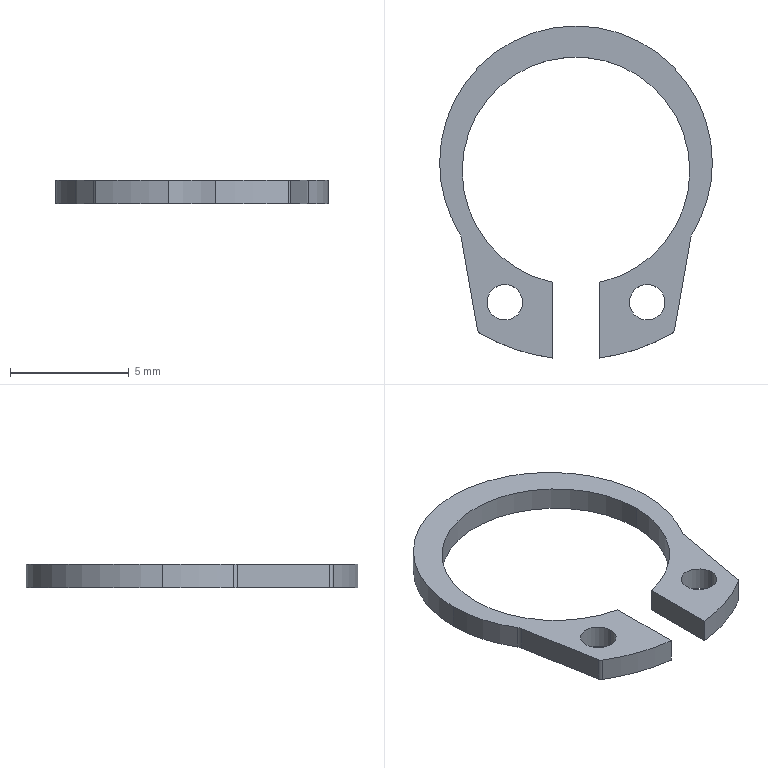Component | SolidWorks | ShaftRetainingRing_10-1 | 1 solid | 22 faces | box 11.5 x 14 x 1 mm | volume 46 mm3 | cylinder 16 | plane 6 | commonest cylinder face diameters 1.5 x4 9.6 x3 11.5 x3 15.9 x2 0.4 x2 1 x2 | material Purchased Part
STEP:
#1=COLOUR_RGB('',0.7922,0.8196,0.9333);
#2=FILL_AREA_STYLE_COLOUR('',#1);
#3=FILL_AREA_STYLE('',(#2));
#4=SURFACE_STYLE_FILL_AREA(#3);
#5=SURFACE_SIDE_STYLE('',(#4));
#6=SURFACE_STYLE_USAGE(.BOTH.,#5);
#7=PRESENTATION_STYLE_ASSIGNMENT((#6));
#8=CARTESIAN_POINT('',(-0.07087,-0.9843,0.9055));
#9=VERTEX_POINT('',#8);
#10=CARTESIAN_POINT('',(0.07874,-1.169,0.9055));
#11=VERTEX_POINT('',#10);
#12=CARTESIAN_POINT('',(0.1181,-0.9843,0.9055));
#13=DIRECTION('',(0.,0.,1.));
#14=DIRECTION('',(-1.,0.,0.));
#15=AXIS2_PLACEMENT_3D('',#12,#13,#14);
#16=CIRCLE('',#15,0.189);
#17=EDGE_CURVE('',#9,#11,#16,.T.);
#18=ORIENTED_EDGE('',*,*,#17,.F.);
#19=CARTESIAN_POINT('',(-0.07087,-0.9843,0.9449));
#20=VERTEX_POINT('',#19);
#21=CARTESIAN_POINT('',(-0.07087,-0.9843,0.9055));
#22=DIRECTION('',(0.,0.,1.));
#23=VECTOR('',#22,39.37);
#24=LINE('',#21,#23);
#25=EDGE_CURVE('',#9,#20,#24,.T.);
#26=ORIENTED_EDGE('',*,*,#25,.T.);
#27=CARTESIAN_POINT('',(0.07874,-1.169,0.9449));
#28=VERTEX_POINT('',#27);
#29=CARTESIAN_POINT('',(0.1181,-0.9843,0.9449));
#30=DIRECTION('',(0.,0.,-1.));
#31=DIRECTION('',(-1.,0.,0.));
#32=AXIS2_PLACEMENT_3D('',#29,#30,#31);
#33=CIRCLE('',#32,0.189);
#34=EDGE_CURVE('',#28,#20,#33,.T.);
#35=ORIENTED_EDGE('',*,*,#34,.F.);
#36=CARTESIAN_POINT('',(0.07874,-1.169,0.9055));
#37=DIRECTION('',(0.,0.,1.));
#38=VECTOR('',#37,39.37);
#39=LINE('',#36,#38);
#40=EDGE_CURVE('',#11,#28,#39,.T.);
#41=ORIENTED_EDGE('',*,*,#40,.F.);
#42=EDGE_LOOP('',(#18,#26,#35,#41));
#43=FACE_OUTER_BOUND('',#42,.T.);
#44=CARTESIAN_POINT('',(0.1181,-0.9843,0.9055));
#45=DIRECTION('',(0.,0.,1.));
#46=DIRECTION('',(1.,0.,0.));
#47=AXIS2_PLACEMENT_3D('',#44,#45,#46);
#48=CYLINDRICAL_SURFACE('',#47,0.189);
#49=ADVANCED_FACE('',(#43),#48,.F.);
#50=ORIENTED_EDGE('',*,*,#25,.F.);
#51=CARTESIAN_POINT('',(0.3071,-0.9843,0.9055));
#52=VERTEX_POINT('',#51);
#53=CARTESIAN_POINT('',(0.1181,-0.9843,0.9055));
#54=DIRECTION('',(0.,0.,1.));
#55=DIRECTION('',(-1.,0.,0.));
#56=AXIS2_PLACEMENT_3D('',#53,#54,#55);
#57=CIRCLE('',#56,0.189);
#58=EDGE_CURVE('',#52,#9,#57,.T.);
#59=ORIENTED_EDGE('',*,*,#58,.F.);
#60=CARTESIAN_POINT('',(0.3071,-0.9843,0.9449));
#61=VERTEX_POINT('',#60);
#62=CARTESIAN_POINT('',(0.3071,-0.9843,0.9055));
#63=DIRECTION('',(0.,0.,1.));
#64=VECTOR('',#63,39.37);
#65=LINE('',#62,#64);
#66=EDGE_CURVE('',#52,#61,#65,.T.);
#67=ORIENTED_EDGE('',*,*,#66,.T.);
#68=CARTESIAN_POINT('',(0.1181,-0.9843,0.9449));
#69=DIRECTION('',(0.,0.,-1.));
#70=DIRECTION('',(-1.,0.,0.));
#71=AXIS2_PLACEMENT_3D('',#68,#69,#70);
#72=CIRCLE('',#71,0.189);
#73=EDGE_CURVE('',#20,#61,#72,.T.);
#74=ORIENTED_EDGE('',*,*,#73,.F.);
#75=EDGE_LOOP('',(#50,#59,#67,#74));
#76=FACE_OUTER_BOUND('',#75,.T.);
#77=CARTESIAN_POINT('',(0.1181,-0.9843,0.9055));
#78=DIRECTION('',(0.,0.,1.));
#79=DIRECTION('',(1.,0.,0.));
#80=AXIS2_PLACEMENT_3D('',#77,#78,#79);
#81=CYLINDRICAL_SURFACE('',#80,0.189);
#82=ADVANCED_FACE('',(#76),#81,.F.);
#83=CARTESIAN_POINT('',(-0.1083,-0.9701,0.9055));
#84=VERTEX_POINT('',#83);
#85=CARTESIAN_POINT('',(0.3445,-0.9701,0.9055));
#86=VERTEX_POINT('',#85);
#87=CARTESIAN_POINT('',(0.1181,-0.9701,0.9055));
#88=DIRECTION('',(0.,0.,-1.));
#89=DIRECTION('',(1.,0.,0.));
#90=AXIS2_PLACEMENT_3D('',#87,#88,#89);
#91=CIRCLE('',#90,0.2264);
#92=EDGE_CURVE('',#84,#86,#91,.T.);
#93=ORIENTED_EDGE('',*,*,#92,.F.);
#94=CARTESIAN_POINT('',(-0.1083,-0.9701,0.9449));
#95=VERTEX_POINT('',#94);
#96=CARTESIAN_POINT('',(-0.1083,-0.9701,0.9055));
#97=DIRECTION('',(0.,0.,1.));
#98=VECTOR('',#97,39.37);
#99=LINE('',#96,#98);
#100=EDGE_CURVE('',#84,#95,#99,.T.);
#101=ORIENTED_EDGE('',*,*,#100,.T.);
#102=CARTESIAN_POINT('',(0.3445,-0.9701,0.9449));
#103=VERTEX_POINT('',#102);
#104=CARTESIAN_POINT('',(0.1181,-0.9701,0.9449));
#105=DIRECTION('',(0.,0.,-1.));
#106=DIRECTION('',(1.,0.,0.));
#107=AXIS2_PLACEMENT_3D('',#104,#105,#106);
#108=CIRCLE('',#107,0.2264);
#109=EDGE_CURVE('',#95,#103,#108,.T.);
#110=ORIENTED_EDGE('',*,*,#109,.T.);
#111=CARTESIAN_POINT('',(0.3445,-0.9701,0.9055));
#112=DIRECTION('',(0.,0.,1.));
#113=VECTOR('',#112,39.37);
#114=LINE('',#111,#113);
#115=EDGE_CURVE('',#86,#103,#114,.T.);
#116=ORIENTED_EDGE('',*,*,#115,.F.);
#117=EDGE_LOOP('',(#93,#101,#110,#116));
#118=FACE_OUTER_BOUND('',#117,.T.);
#119=CARTESIAN_POINT('',(0.1181,-0.9701,0.9055));
#120=DIRECTION('',(0.,0.,1.));
#121=DIRECTION('',(1.,0.,0.));
#122=AXIS2_PLACEMENT_3D('',#119,#120,#121);
#123=CYLINDRICAL_SURFACE('',#122,0.2264);
#124=ADVANCED_FACE('',(#118),#123,.T.);
#125=CARTESIAN_POINT('',(0.3113,-1.088,0.9055));
#126=VERTEX_POINT('',#125);
#127=CARTESIAN_POINT('',(0.1181,-0.9701,0.9055));
#128=DIRECTION('',(0.,0.,-1.));
#129=DIRECTION('',(1.,0.,0.));
#130=AXIS2_PLACEMENT_3D('',#127,#128,#129);
#131=CIRCLE('',#130,0.2264);
#132=EDGE_CURVE('',#86,#126,#131,.T.);
#133=ORIENTED_EDGE('',*,*,#132,.F.);
#134=ORIENTED_EDGE('',*,*,#115,.T.);
#135=CARTESIAN_POINT('',(0.3113,-1.088,0.9449));
#136=VERTEX_POINT('',#135);
#137=CARTESIAN_POINT('',(0.1181,-0.9701,0.9449));
#138=DIRECTION('',(0.,0.,-1.));
#139=DIRECTION('',(1.,0.,0.));
#140=AXIS2_PLACEMENT_3D('',#137,#138,#139);
#141=CIRCLE('',#140,0.2264);
#142=EDGE_CURVE('',#103,#136,#141,.T.);
#143=ORIENTED_EDGE('',*,*,#142,.T.);
#144=CARTESIAN_POINT('',(0.3113,-1.088,0.9055));
#145=DIRECTION('',(0.,0.,-1.));
#146=VECTOR('',#145,39.37);
#147=LINE('',#144,#146);
#148=EDGE_CURVE('',#136,#126,#147,.T.);
#149=ORIENTED_EDGE('',*,*,#148,.T.);
#150=EDGE_LOOP('',(#133,#134,#143,#149));
#151=FACE_OUTER_BOUND('',#150,.T.);
#152=CARTESIAN_POINT('',(0.1181,-0.9701,0.9055));
#153=DIRECTION('',(0.,0.,1.));
#154=DIRECTION('',(1.,0.,0.));
#155=AXIS2_PLACEMENT_3D('',#152,#153,#154);
#156=CYLINDRICAL_SURFACE('',#155,0.2264);
#157=ADVANCED_FACE('',(#151),#156,.T.);
#158=CARTESIAN_POINT('',(-0.02953,-1.202,0.9055));
#159=VERTEX_POINT('',#158);
#160=CARTESIAN_POINT('',(0.02953,-1.202,0.9055));
#161=VERTEX_POINT('',#160);
#162=CARTESIAN_POINT('',(-0.,-1.202,0.9055));
#163=DIRECTION('',(0.,0.,1.));
#164=DIRECTION('',(1.,0.,0.));
#165=AXIS2_PLACEMENT_3D('',#162,#163,#164);
#166=CIRCLE('',#165,0.02953);
#167=EDGE_CURVE('',#159,#161,#166,.T.);
#168=ORIENTED_EDGE('',*,*,#167,.F.);
#169=CARTESIAN_POINT('',(-0.02953,-1.202,0.9449));
#170=VERTEX_POINT('',#169);
#171=CARTESIAN_POINT('',(-0.02953,-1.202,0.9055));
#172=DIRECTION('',(0.,0.,1.));
#173=VECTOR('',#172,39.37);
#174=LINE('',#171,#173);
#175=EDGE_CURVE('',#159,#170,#174,.T.);
#176=ORIENTED_EDGE('',*,*,#175,.T.);
#177=CARTESIAN_POINT('',(0.02953,-1.202,0.9449));
#178=VERTEX_POINT('',#177);
#179=CARTESIAN_POINT('',(-0.,-1.202,0.9449));
#180=DIRECTION('',(0.,0.,-1.));
#181=DIRECTION('',(1.,0.,0.));
#182=AXIS2_PLACEMENT_3D('',#179,#180,#181);
#183=CIRCLE('',#182,0.02953);
#184=EDGE_CURVE('',#178,#170,#183,.T.);
#185=ORIENTED_EDGE('',*,*,#184,.F.);
#186=CARTESIAN_POINT('',(0.02953,-1.202,0.9055));
#187=DIRECTION('',(0.,0.,1.));
#188=VECTOR('',#187,39.37);
#189=LINE('',#186,#188);
#190=EDGE_CURVE('',#161,#178,#189,.T.);
#191=ORIENTED_EDGE('',*,*,#190,.F.);
#192=EDGE_LOOP('',(#168,#176,#185,#191));
#193=FACE_OUTER_BOUND('',#192,.T.);
#194=CARTESIAN_POINT('',(-0.,-1.202,0.9055));
#195=DIRECTION('',(0.,0.,1.));
#196=DIRECTION('',(1.,0.,0.));
#197=AXIS2_PLACEMENT_3D('',#194,#195,#196);
#198=CYLINDRICAL_SURFACE('',#197,0.02953);
#199=ADVANCED_FACE('',(#193),#198,.F.);
#200=CARTESIAN_POINT('',(0.2067,-1.202,0.9055));
#201=VERTEX_POINT('',#200);
#202=CARTESIAN_POINT('',(0.2657,-1.202,0.9055));
#203=VERTEX_POINT('',#202);
#204=CARTESIAN_POINT('',(0.2362,-1.202,0.9055));
#205=DIRECTION('',(0.,0.,1.));
#206=DIRECTION('',(1.,0.,0.));
#207=AXIS2_PLACEMENT_3D('',#204,#205,#206);
#208=CIRCLE('',#207,0.02953);
#209=EDGE_CURVE('',#201,#203,#208,.T.);
#210=ORIENTED_EDGE('',*,*,#209,.F.);
#211=CARTESIAN_POINT('',(0.2067,-1.202,0.9449));
#212=VERTEX_POINT('',#211);
#213=CARTESIAN_POINT('',(0.2067,-1.202,0.9055));
#214=DIRECTION('',(0.,0.,1.));
#215=VECTOR('',#214,39.37);
#216=LINE('',#213,#215);
#217=EDGE_CURVE('',#201,#212,#216,.T.);
#218=ORIENTED_EDGE('',*,*,#217,.T.);
#219=CARTESIAN_POINT('',(0.2657,-1.202,0.9449));
#220=VERTEX_POINT('',#219);
#221=CARTESIAN_POINT('',(0.2362,-1.202,0.9449));
#222=DIRECTION('',(0.,0.,-1.));
#223=DIRECTION('',(1.,0.,0.));
#224=AXIS2_PLACEMENT_3D('',#221,#222,#223);
#225=CIRCLE('',#224,0.02953);
#226=EDGE_CURVE('',#220,#212,#225,.T.);
#227=ORIENTED_EDGE('',*,*,#226,.F.);
#228=CARTESIAN_POINT('',(0.2657,-1.202,0.9055));
#229=DIRECTION('',(0.,0.,1.));
#230=VECTOR('',#229,39.37);
#231=LINE('',#228,#230);
#232=EDGE_CURVE('',#203,#220,#231,.T.);
#233=ORIENTED_EDGE('',*,*,#232,.F.);
#234=EDGE_LOOP('',(#210,#218,#227,#233));
#235=FACE_OUTER_BOUND('',#234,.T.);
#236=CARTESIAN_POINT('',(0.2362,-1.202,0.9055));
#237=DIRECTION('',(0.,0.,1.));
#238=DIRECTION('',(1.,0.,0.));
#239=AXIS2_PLACEMENT_3D('',#236,#237,#238);
#240=CYLINDRICAL_SURFACE('',#239,0.02953);
#241=ADVANCED_FACE('',(#235),#240,.F.);
#242=CARTESIAN_POINT('',(0.1575,-1.169,0.9055));
#243=VERTEX_POINT('',#242);
#244=CARTESIAN_POINT('',(0.1181,-0.9843,0.9055));
#245=DIRECTION('',(0.,0.,1.));
#246=DIRECTION('',(-1.,0.,0.));
#247=AXIS2_PLACEMENT_3D('',#244,#245,#246);
#248=CIRCLE('',#247,0.189);
#249=EDGE_CURVE('',#243,#52,#248,.T.);
#250=ORIENTED_EDGE('',*,*,#249,.T.);
#251=ORIENTED_EDGE('',*,*,#58,.T.);
#252=ORIENTED_EDGE('',*,*,#17,.T.);
#253=CARTESIAN_POINT('',(0.07874,-1.295,0.9055));
#254=VERTEX_POINT('',#253);
#255=CARTESIAN_POINT('',(0.07874,-0.9843,0.9055));
#256=DIRECTION('',(0.,-1.,0.));
#257=VECTOR('',#256,39.37);
#258=LINE('',#255,#257);
#259=EDGE_CURVE('',#11,#254,#258,.T.);
#260=ORIENTED_EDGE('',*,*,#259,.T.);
#261=CARTESIAN_POINT('',(-0.04181,-1.253,0.9055));
#262=VERTEX_POINT('',#261);
#263=CARTESIAN_POINT('',(0.1181,-0.9843,0.9055));
#264=DIRECTION('',(0.,0.,-1.));
#265=DIRECTION('',(1.,-0.,0.));
#266=AXIS2_PLACEMENT_3D('',#263,#264,#265);
#267=CIRCLE('',#266,0.313);
#268=EDGE_CURVE('',#254,#262,#267,.T.);
#269=ORIENTED_EDGE('',*,*,#268,.T.);
#270=CARTESIAN_POINT('',(-0.04554,-1.248,0.9055));
#271=VERTEX_POINT('',#270);
#272=CARTESIAN_POINT('',(-0.03779,-1.247,0.9055));
#273=DIRECTION('',(0.,0.,-1.));
#274=DIRECTION('',(1.,-0.,0.));
#275=AXIS2_PLACEMENT_3D('',#272,#273,#274);
#276=CIRCLE('',#275,0.007874);
#277=EDGE_CURVE('',#262,#271,#276,.T.);
#278=ORIENTED_EDGE('',*,*,#277,.T.);
#279=CARTESIAN_POINT('',(-0.07253,-1.095,0.9055));
#280=VERTEX_POINT('',#279);
#281=CARTESIAN_POINT('',(-0.04554,-1.248,0.9055));
#282=DIRECTION('',(-0.1736,0.9848,0.));
#283=VECTOR('',#282,39.37);
#284=LINE('',#281,#283);
#285=EDGE_CURVE('',#271,#280,#284,.T.);
#286=ORIENTED_EDGE('',*,*,#285,.T.);
#287=CARTESIAN_POINT('',(-0.07511,-1.088,0.9055));
#288=VERTEX_POINT('',#287);
#289=CARTESIAN_POINT('',(-0.09191,-1.098,0.9055));
#290=DIRECTION('',(0.,0.,1.));
#291=DIRECTION('',(1.,0.,0.));
#292=AXIS2_PLACEMENT_3D('',#289,#290,#291);
#293=CIRCLE('',#292,0.01969);
#294=EDGE_CURVE('',#280,#288,#293,.T.);
#295=ORIENTED_EDGE('',*,*,#294,.T.);
#296=CARTESIAN_POINT('',(0.1181,-0.9701,0.9055));
#297=DIRECTION('',(0.,0.,-1.));
#298=DIRECTION('',(1.,0.,0.));
#299=AXIS2_PLACEMENT_3D('',#296,#297,#298);
#300=CIRCLE('',#299,0.2264);
#301=EDGE_CURVE('',#288,#84,#300,.T.);
#302=ORIENTED_EDGE('',*,*,#301,.T.);
#303=ORIENTED_EDGE('',*,*,#92,.T.);
#304=ORIENTED_EDGE('',*,*,#132,.T.);
#305=CARTESIAN_POINT('',(0.3087,-1.095,0.9055));
#306=VERTEX_POINT('',#305);
#307=CARTESIAN_POINT('',(0.3281,-1.098,0.9055));
#308=DIRECTION('',(0.,0.,1.));
#309=DIRECTION('',(1.,0.,0.));
#310=AXIS2_PLACEMENT_3D('',#307,#308,#309);
#311=CIRCLE('',#310,0.01969);
#312=EDGE_CURVE('',#126,#306,#311,.T.);
#313=ORIENTED_EDGE('',*,*,#312,.T.);
#314=CARTESIAN_POINT('',(0.2818,-1.248,0.9055));
#315=VERTEX_POINT('',#314);
#316=CARTESIAN_POINT('',(0.3087,-1.095,0.9055));
#317=DIRECTION('',(-0.1736,-0.9848,0.));
#318=VECTOR('',#317,39.37);
#319=LINE('',#316,#318);
#320=EDGE_CURVE('',#306,#315,#319,.T.);
#321=ORIENTED_EDGE('',*,*,#320,.T.);
#322=CARTESIAN_POINT('',(0.278,-1.253,0.9055));
#323=VERTEX_POINT('',#322);
#324=CARTESIAN_POINT('',(0.274,-1.247,0.9055));
#325=DIRECTION('',(0.,0.,-1.));
#326=DIRECTION('',(1.,0.,0.));
#327=AXIS2_PLACEMENT_3D('',#324,#325,#326);
#328=CIRCLE('',#327,0.007874);
#329=EDGE_CURVE('',#315,#323,#328,.T.);
#330=ORIENTED_EDGE('',*,*,#329,.T.);
#331=CARTESIAN_POINT('',(0.1575,-1.295,0.9055));
#332=VERTEX_POINT('',#331);
#333=CARTESIAN_POINT('',(0.1181,-0.9843,0.9055));
#334=DIRECTION('',(0.,0.,-1.));
#335=DIRECTION('',(1.,0.,0.));
#336=AXIS2_PLACEMENT_3D('',#333,#334,#335);
#337=CIRCLE('',#336,0.313);
#338=EDGE_CURVE('',#323,#332,#337,.T.);
#339=ORIENTED_EDGE('',*,*,#338,.T.);
#340=CARTESIAN_POINT('',(0.1575,-0.9843,0.9055));
#341=DIRECTION('',(0.,1.,0.));
#342=VECTOR('',#341,39.37);
#343=LINE('',#340,#342);
#344=EDGE_CURVE('',#332,#243,#343,.T.);
#345=ORIENTED_EDGE('',*,*,#344,.T.);
#346=EDGE_LOOP('',(#250,#251,#252,#260,#269,#278,#286,#295,#302,#303,#304,#313,#321,#330,#339,#345));
#347=FACE_OUTER_BOUND('',#346,.T.);
#348=CARTESIAN_POINT('',(-0.,-1.202,0.9055));
#349=DIRECTION('',(0.,0.,1.));
#350=DIRECTION('',(1.,0.,0.));
#351=AXIS2_PLACEMENT_3D('',#348,#349,#350);
#352=CIRCLE('',#351,0.02953);
#353=EDGE_CURVE('',#161,#159,#352,.T.);
#354=ORIENTED_EDGE('',*,*,#353,.T.);
#355=ORIENTED_EDGE('',*,*,#167,.T.);
#356=EDGE_LOOP('',(#354,#355));
#357=FACE_BOUND('',#356,.T.);
#358=CARTESIAN_POINT('',(0.2362,-1.202,0.9055));
#359=DIRECTION('',(0.,0.,1.));
#360=DIRECTION('',(1.,0.,0.));
#361=AXIS2_PLACEMENT_3D('',#358,#359,#360);
#362=CIRCLE('',#361,0.02953);
#363=EDGE_CURVE('',#203,#201,#362,.T.);
#364=ORIENTED_EDGE('',*,*,#363,.T.);
#365=ORIENTED_EDGE('',*,*,#209,.T.);
#366=EDGE_LOOP('',(#364,#365));
#367=FACE_BOUND('',#366,.T.);
#368=CARTESIAN_POINT('',(0.1181,-0.9843,0.9055));
#369=DIRECTION('',(0.,0.,-1.));
#370=DIRECTION('',(-1.,0.,0.));
#371=AXIS2_PLACEMENT_3D('',#368,#369,#370);
#372=PLANE('',#371);
#373=ADVANCED_FACE('',(#347,#357,#367),#372,.T.);
#374=ORIENTED_EDGE('',*,*,#259,.F.);
#375=ORIENTED_EDGE('',*,*,#40,.T.);
#376=CARTESIAN_POINT('',(0.07874,-1.295,0.9449));
#377=VERTEX_POINT('',#376);
#378=CARTESIAN_POINT('',(0.07874,-1.163,0.9449));
#379=DIRECTION('',(0.,-1.,0.));
#380=VECTOR('',#379,39.37);
#381=LINE('',#378,#380);
#382=EDGE_CURVE('',#28,#377,#381,.T.);
#383=ORIENTED_EDGE('',*,*,#382,.T.);
#384=CARTESIAN_POINT('',(0.07874,-1.295,0.9055));
#385=DIRECTION('',(0.,0.,-1.));
#386=VECTOR('',#385,39.37);
#387=LINE('',#384,#386);
#388=EDGE_CURVE('',#377,#254,#387,.T.);
#389=ORIENTED_EDGE('',*,*,#388,.T.);
#390=EDGE_LOOP('',(#374,#375,#383,#389));
#391=FACE_OUTER_BOUND('',#390,.T.);
#392=CARTESIAN_POINT('',(0.07874,-1.163,0.9055));
#393=DIRECTION('',(1.,0.,0.));
#394=DIRECTION('',(-0.,1.,0.));
#395=AXIS2_PLACEMENT_3D('',#392,#393,#394);
#396=PLANE('',#395);
#397=ADVANCED_FACE('',(#391),#396,.T.);
#398=ORIENTED_EDGE('',*,*,#66,.F.);
#399=ORIENTED_EDGE('',*,*,#249,.F.);
#400=CARTESIAN_POINT('',(0.1575,-1.169,0.9449));
#401=VERTEX_POINT('',#400);
#402=CARTESIAN_POINT('',(0.1575,-1.169,0.9055));
#403=DIRECTION('',(0.,0.,-1.));
#404=VECTOR('',#403,39.37);
#405=LINE('',#402,#404);
#406=EDGE_CURVE('',#401,#243,#405,.T.);
#407=ORIENTED_EDGE('',*,*,#406,.F.);
#408=CARTESIAN_POINT('',(0.1181,-0.9843,0.9449));
#409=DIRECTION('',(0.,0.,-1.));
#410=DIRECTION('',(-1.,0.,0.));
#411=AXIS2_PLACEMENT_3D('',#408,#409,#410);
#412=CIRCLE('',#411,0.189);
#413=EDGE_CURVE('',#61,#401,#412,.T.);
#414=ORIENTED_EDGE('',*,*,#413,.F.);
#415=EDGE_LOOP('',(#398,#399,#407,#414));
#416=FACE_OUTER_BOUND('',#415,.T.);
#417=CARTESIAN_POINT('',(0.1181,-0.9843,0.9055));
#418=DIRECTION('',(0.,0.,1.));
#419=DIRECTION('',(1.,0.,0.));
#420=AXIS2_PLACEMENT_3D('',#417,#418,#419);
#421=CYLINDRICAL_SURFACE('',#420,0.189);
#422=ADVANCED_FACE('',(#416),#421,.F.);
#423=ORIENTED_EDGE('',*,*,#344,.F.);
#424=CARTESIAN_POINT('',(0.1575,-1.295,0.9449));
#425=VERTEX_POINT('',#424);
#426=CARTESIAN_POINT('',(0.1575,-1.295,0.9055));
#427=DIRECTION('',(0.,0.,1.));
#428=VECTOR('',#427,39.37);
#429=LINE('',#426,#428);
#430=EDGE_CURVE('',#332,#425,#429,.T.);
#431=ORIENTED_EDGE('',*,*,#430,.T.);
#432=CARTESIAN_POINT('',(0.1575,-1.163,0.9449));
#433=DIRECTION('',(0.,1.,0.));
#434=VECTOR('',#433,39.37);
#435=LINE('',#432,#434);
#436=EDGE_CURVE('',#425,#401,#435,.T.);
#437=ORIENTED_EDGE('',*,*,#436,.T.);
#438=ORIENTED_EDGE('',*,*,#406,.T.);
#439=EDGE_LOOP('',(#423,#431,#437,#438));
#440=FACE_OUTER_BOUND('',#439,.T.);
#441=CARTESIAN_POINT('',(0.1575,-1.163,0.9055));
#442=DIRECTION('',(-1.,0.,0.));
#443=DIRECTION('',(-0.,-1.,0.));
#444=AXIS2_PLACEMENT_3D('',#441,#442,#443);
#445=PLANE('',#444);
#446=ADVANCED_FACE('',(#440),#445,.T.);
#447=CARTESIAN_POINT('',(0.278,-1.253,0.9449));
#448=VERTEX_POINT('',#447);
#449=CARTESIAN_POINT('',(0.1181,-0.9843,0.9449));
#450=DIRECTION('',(0.,0.,-1.));
#451=DIRECTION('',(1.,0.,0.));
#452=AXIS2_PLACEMENT_3D('',#449,#450,#451);
#453=CIRCLE('',#452,0.313);
#454=EDGE_CURVE('',#448,#425,#453,.T.);
#455=ORIENTED_EDGE('',*,*,#454,.T.);
#456=ORIENTED_EDGE('',*,*,#430,.F.);
#457=ORIENTED_EDGE('',*,*,#338,.F.);
#458=CARTESIAN_POINT('',(0.278,-1.253,0.9055));
#459=DIRECTION('',(0.,0.,1.));
#460=VECTOR('',#459,39.37);
#461=LINE('',#458,#460);
#462=EDGE_CURVE('',#323,#448,#461,.T.);
#463=ORIENTED_EDGE('',*,*,#462,.T.);
#464=EDGE_LOOP('',(#455,#456,#457,#463));
#465=FACE_OUTER_BOUND('',#464,.T.);
#466=CARTESIAN_POINT('',(0.1181,-0.9843,0.9055));
#467=DIRECTION('',(0.,0.,1.));
#468=DIRECTION('',(1.,0.,0.));
#469=AXIS2_PLACEMENT_3D('',#466,#467,#468);
#470=CYLINDRICAL_SURFACE('',#469,0.313);
#471=ADVANCED_FACE('',(#465),#470,.T.);
#472=CARTESIAN_POINT('',(0.2818,-1.248,0.9449));
#473=VERTEX_POINT('',#472);
#474=CARTESIAN_POINT('',(0.274,-1.247,0.9449));
#475=DIRECTION('',(0.,0.,-1.));
#476=DIRECTION('',(1.,0.,0.));
#477=AXIS2_PLACEMENT_3D('',#474,#475,#476);
#478=CIRCLE('',#477,0.007874);
#479=EDGE_CURVE('',#473,#448,#478,.T.);
#480=ORIENTED_EDGE('',*,*,#479,.T.);
#481=ORIENTED_EDGE('',*,*,#462,.F.);
#482=ORIENTED_EDGE('',*,*,#329,.F.);
#483=CARTESIAN_POINT('',(0.2818,-1.248,0.9055));
#484=DIRECTION('',(0.,0.,1.));
#485=VECTOR('',#484,39.37);
#486=LINE('',#483,#485);
#487=EDGE_CURVE('',#315,#473,#486,.T.);
#488=ORIENTED_EDGE('',*,*,#487,.T.);
#489=EDGE_LOOP('',(#480,#481,#482,#488));
#490=FACE_OUTER_BOUND('',#489,.T.);
#491=CARTESIAN_POINT('',(0.274,-1.247,0.9055));
#492=DIRECTION('',(0.,0.,1.));
#493=DIRECTION('',(1.,0.,0.));
#494=AXIS2_PLACEMENT_3D('',#491,#492,#493);
#495=CYLINDRICAL_SURFACE('',#494,0.007874);
#496=ADVANCED_FACE('',(#490),#495,.T.);
#497=CARTESIAN_POINT('',(0.3087,-1.095,0.9449));
#498=VERTEX_POINT('',#497);
#499=CARTESIAN_POINT('',(0.3094,-1.091,0.9449));
#500=DIRECTION('',(-0.1736,-0.9848,0.));
#501=VECTOR('',#500,39.37);
#502=LINE('',#499,#501);
#503=EDGE_CURVE('',#498,#473,#502,.T.);
#504=ORIENTED_EDGE('',*,*,#503,.T.);
#505=ORIENTED_EDGE('',*,*,#487,.F.);
#506=ORIENTED_EDGE('',*,*,#320,.F.);
#507=CARTESIAN_POINT('',(0.3087,-1.095,0.9055));
#508=DIRECTION('',(0.,0.,1.));
#509=VECTOR('',#508,39.37);
#510=LINE('',#507,#509);
#511=EDGE_CURVE('',#306,#498,#510,.T.);
#512=ORIENTED_EDGE('',*,*,#511,.T.);
#513=EDGE_LOOP('',(#504,#505,#506,#512));
#514=FACE_OUTER_BOUND('',#513,.T.);
#515=CARTESIAN_POINT('',(0.3094,-1.091,0.9055));
#516=DIRECTION('',(0.9848,-0.1736,0.));
#517=DIRECTION('',(0.1736,0.9848,0.));
#518=AXIS2_PLACEMENT_3D('',#515,#516,#517);
#519=PLANE('',#518);
#520=ADVANCED_FACE('',(#514),#519,.T.);
#521=ORIENTED_EDGE('',*,*,#148,.F.);
#522=CARTESIAN_POINT('',(0.3281,-1.098,0.9449));
#523=DIRECTION('',(0.,0.,-1.));
#524=DIRECTION('',(1.,0.,0.));
#525=AXIS2_PLACEMENT_3D('',#522,#523,#524);
#526=CIRCLE('',#525,0.01969);
#527=EDGE_CURVE('',#498,#136,#526,.T.);
#528=ORIENTED_EDGE('',*,*,#527,.F.);
#529=ORIENTED_EDGE('',*,*,#511,.F.);
#530=ORIENTED_EDGE('',*,*,#312,.F.);
#531=EDGE_LOOP('',(#521,#528,#529,#530));
#532=FACE_OUTER_BOUND('',#531,.T.);
#533=CARTESIAN_POINT('',(0.3281,-1.098,0.9055));
#534=DIRECTION('',(0.,0.,1.));
#535=DIRECTION('',(1.,0.,0.));
#536=AXIS2_PLACEMENT_3D('',#533,#534,#535);
#537=CYLINDRICAL_SURFACE('',#536,0.01969);
#538=ADVANCED_FACE('',(#532),#537,.F.);
#539=ORIENTED_EDGE('',*,*,#100,.F.);
#540=ORIENTED_EDGE('',*,*,#301,.F.);
#541=CARTESIAN_POINT('',(-0.07511,-1.088,0.9449));
#542=VERTEX_POINT('',#541);
#543=CARTESIAN_POINT('',(-0.07511,-1.088,0.9055));
#544=DIRECTION('',(0.,0.,1.));
#545=VECTOR('',#544,39.37);
#546=LINE('',#543,#545);
#547=EDGE_CURVE('',#288,#542,#546,.T.);
#548=ORIENTED_EDGE('',*,*,#547,.T.);
#549=CARTESIAN_POINT('',(0.1181,-0.9701,0.9449));
#550=DIRECTION('',(0.,0.,-1.));
#551=DIRECTION('',(1.,0.,0.));
#552=AXIS2_PLACEMENT_3D('',#549,#550,#551);
#553=CIRCLE('',#552,0.2264);
#554=EDGE_CURVE('',#542,#95,#553,.T.);
#555=ORIENTED_EDGE('',*,*,#554,.T.);
#556=EDGE_LOOP('',(#539,#540,#548,#555));
#557=FACE_OUTER_BOUND('',#556,.T.);
#558=CARTESIAN_POINT('',(0.1181,-0.9701,0.9055));
#559=DIRECTION('',(0.,0.,1.));
#560=DIRECTION('',(1.,0.,0.));
#561=AXIS2_PLACEMENT_3D('',#558,#559,#560);
#562=CYLINDRICAL_SURFACE('',#561,0.2264);
#563=ADVANCED_FACE('',(#557),#562,.T.);
#564=CARTESIAN_POINT('',(-0.07253,-1.095,0.9449));
#565=VERTEX_POINT('',#564);
#566=CARTESIAN_POINT('',(-0.07253,-1.095,0.9055));
#567=DIRECTION('',(0.,0.,-1.));
#568=VECTOR('',#567,39.37);
#569=LINE('',#566,#568);
#570=EDGE_CURVE('',#565,#280,#569,.T.);
#571=ORIENTED_EDGE('',*,*,#570,.F.);
#572=CARTESIAN_POINT('',(-0.09191,-1.098,0.9449));
#573=DIRECTION('',(0.,0.,-1.));
#574=DIRECTION('',(1.,0.,0.));
#575=AXIS2_PLACEMENT_3D('',#572,#573,#574);
#576=CIRCLE('',#575,0.01969);
#577=EDGE_CURVE('',#542,#565,#576,.T.);
#578=ORIENTED_EDGE('',*,*,#577,.F.);
#579=ORIENTED_EDGE('',*,*,#547,.F.);
#580=ORIENTED_EDGE('',*,*,#294,.F.);
#581=EDGE_LOOP('',(#571,#578,#579,#580));
#582=FACE_OUTER_BOUND('',#581,.T.);
#583=CARTESIAN_POINT('',(-0.09191,-1.098,0.9055));
#584=DIRECTION('',(0.,0.,1.));
#585=DIRECTION('',(1.,0.,0.));
#586=AXIS2_PLACEMENT_3D('',#583,#584,#585);
#587=CYLINDRICAL_SURFACE('',#586,0.01969);
#588=ADVANCED_FACE('',(#582),#587,.F.);
#589=ORIENTED_EDGE('',*,*,#285,.F.);
#590=CARTESIAN_POINT('',(-0.04554,-1.248,0.9449));
#591=VERTEX_POINT('',#590);
#592=CARTESIAN_POINT('',(-0.04554,-1.248,0.9055));
#593=DIRECTION('',(0.,0.,1.));
#594=VECTOR('',#593,39.37);
#595=LINE('',#592,#594);
#596=EDGE_CURVE('',#271,#591,#595,.T.);
#597=ORIENTED_EDGE('',*,*,#596,.T.);
#598=CARTESIAN_POINT('',(-0.07319,-1.091,0.9449));
#599=DIRECTION('',(-0.1736,0.9848,0.));
#600=VECTOR('',#599,39.37);
#601=LINE('',#598,#600);
#602=EDGE_CURVE('',#591,#565,#601,.T.);
#603=ORIENTED_EDGE('',*,*,#602,.T.);
#604=ORIENTED_EDGE('',*,*,#570,.T.);
#605=EDGE_LOOP('',(#589,#597,#603,#604));
#606=FACE_OUTER_BOUND('',#605,.T.);
#607=CARTESIAN_POINT('',(-0.07319,-1.091,0.9055));
#608=DIRECTION('',(-0.9848,-0.1736,0.));
#609=DIRECTION('',(0.1736,-0.9848,0.));
#610=AXIS2_PLACEMENT_3D('',#607,#608,#609);
#611=PLANE('',#610);
#612=ADVANCED_FACE('',(#606),#611,.T.);
#613=CARTESIAN_POINT('',(-0.04181,-1.253,0.9449));
#614=VERTEX_POINT('',#613);
#615=CARTESIAN_POINT('',(-0.03779,-1.247,0.9449));
#616=DIRECTION('',(0.,0.,-1.));
#617=DIRECTION('',(1.,-0.,0.));
#618=AXIS2_PLACEMENT_3D('',#615,#616,#617);
#619=CIRCLE('',#618,0.007874);
#620=EDGE_CURVE('',#614,#591,#619,.T.);
#621=ORIENTED_EDGE('',*,*,#620,.T.);
#622=ORIENTED_EDGE('',*,*,#596,.F.);
#623=ORIENTED_EDGE('',*,*,#277,.F.);
#624=CARTESIAN_POINT('',(-0.04181,-1.253,0.9055));
#625=DIRECTION('',(0.,0.,1.));
#626=VECTOR('',#625,39.37);
#627=LINE('',#624,#626);
#628=EDGE_CURVE('',#262,#614,#627,.T.);
#629=ORIENTED_EDGE('',*,*,#628,.T.);
#630=EDGE_LOOP('',(#621,#622,#623,#629));
#631=FACE_OUTER_BOUND('',#630,.T.);
#632=CARTESIAN_POINT('',(-0.03779,-1.247,0.9055));
#633=DIRECTION('',(0.,0.,1.));
#634=DIRECTION('',(1.,0.,0.));
#635=AXIS2_PLACEMENT_3D('',#632,#633,#634);
#636=CYLINDRICAL_SURFACE('',#635,0.007874);
#637=ADVANCED_FACE('',(#631),#636,.T.);
#638=ORIENTED_EDGE('',*,*,#268,.F.);
#639=ORIENTED_EDGE('',*,*,#388,.F.);
#640=CARTESIAN_POINT('',(0.1181,-0.9843,0.9449));
#641=DIRECTION('',(0.,0.,-1.));
#642=DIRECTION('',(1.,-0.,0.));
#643=AXIS2_PLACEMENT_3D('',#640,#641,#642);
#644=CIRCLE('',#643,0.313);
#645=EDGE_CURVE('',#377,#614,#644,.T.);
#646=ORIENTED_EDGE('',*,*,#645,.T.);
#647=ORIENTED_EDGE('',*,*,#628,.F.);
#648=EDGE_LOOP('',(#638,#639,#646,#647));
#649=FACE_OUTER_BOUND('',#648,.T.);
#650=CARTESIAN_POINT('',(0.1181,-0.9843,0.9055));
#651=DIRECTION('',(0.,0.,1.));
#652=DIRECTION('',(1.,0.,0.));
#653=AXIS2_PLACEMENT_3D('',#650,#651,#652);
#654=CYLINDRICAL_SURFACE('',#653,0.313);
#655=ADVANCED_FACE('',(#649),#654,.T.);
#656=ORIENTED_EDGE('',*,*,#175,.F.);
#657=ORIENTED_EDGE('',*,*,#353,.F.);
#658=ORIENTED_EDGE('',*,*,#190,.T.);
#659=CARTESIAN_POINT('',(-0.,-1.202,0.9449));
#660=DIRECTION('',(0.,0.,-1.));
#661=DIRECTION('',(1.,0.,0.));
#662=AXIS2_PLACEMENT_3D('',#659,#660,#661);
#663=CIRCLE('',#662,0.02953);
#664=EDGE_CURVE('',#170,#178,#663,.T.);
#665=ORIENTED_EDGE('',*,*,#664,.F.);
#666=EDGE_LOOP('',(#656,#657,#658,#665));
#667=FACE_OUTER_BOUND('',#666,.T.);
#668=CARTESIAN_POINT('',(-0.,-1.202,0.9055));
#669=DIRECTION('',(0.,0.,1.));
#670=DIRECTION('',(1.,0.,0.));
#671=AXIS2_PLACEMENT_3D('',#668,#669,#670);
#672=CYLINDRICAL_SURFACE('',#671,0.02953);
#673=ADVANCED_FACE('',(#667),#672,.F.);
#674=ORIENTED_EDGE('',*,*,#217,.F.);
#675=ORIENTED_EDGE('',*,*,#363,.F.);
#676=ORIENTED_EDGE('',*,*,#232,.T.);
#677=CARTESIAN_POINT('',(0.2362,-1.202,0.9449));
#678=DIRECTION('',(0.,0.,-1.));
#679=DIRECTION('',(1.,0.,0.));
#680=AXIS2_PLACEMENT_3D('',#677,#678,#679);
#681=CIRCLE('',#680,0.02953);
#682=EDGE_CURVE('',#212,#220,#681,.T.);
#683=ORIENTED_EDGE('',*,*,#682,.F.);
#684=EDGE_LOOP('',(#674,#675,#676,#683));
#685=FACE_OUTER_BOUND('',#684,.T.);
#686=CARTESIAN_POINT('',(0.2362,-1.202,0.9055));
#687=DIRECTION('',(0.,0.,1.));
#688=DIRECTION('',(1.,0.,0.));
#689=AXIS2_PLACEMENT_3D('',#686,#687,#688);
#690=CYLINDRICAL_SURFACE('',#689,0.02953);
#691=ADVANCED_FACE('',(#685),#690,.F.);
#692=ORIENTED_EDGE('',*,*,#554,.F.);
#693=ORIENTED_EDGE('',*,*,#577,.T.);
#694=ORIENTED_EDGE('',*,*,#602,.F.);
#695=ORIENTED_EDGE('',*,*,#620,.F.);
#696=ORIENTED_EDGE('',*,*,#645,.F.);
#697=ORIENTED_EDGE('',*,*,#382,.F.);
#698=ORIENTED_EDGE('',*,*,#34,.T.);
#699=ORIENTED_EDGE('',*,*,#73,.T.);
#700=ORIENTED_EDGE('',*,*,#413,.T.);
#701=ORIENTED_EDGE('',*,*,#436,.F.);
#702=ORIENTED_EDGE('',*,*,#454,.F.);
#703=ORIENTED_EDGE('',*,*,#479,.F.);
#704=ORIENTED_EDGE('',*,*,#503,.F.);
#705=ORIENTED_EDGE('',*,*,#527,.T.);
#706=ORIENTED_EDGE('',*,*,#142,.F.);
#707=ORIENTED_EDGE('',*,*,#109,.F.);
#708=EDGE_LOOP('',(#692,#693,#694,#695,#696,#697,#698,#699,#700,#701,#702,#703,#704,#705,#706,#707));
#709=FACE_OUTER_BOUND('',#708,.T.);
#710=ORIENTED_EDGE('',*,*,#184,.T.);
#711=ORIENTED_EDGE('',*,*,#664,.T.);
#712=EDGE_LOOP('',(#710,#711));
#713=FACE_BOUND('',#712,.T.);
#714=ORIENTED_EDGE('',*,*,#226,.T.);
#715=ORIENTED_EDGE('',*,*,#682,.T.);
#716=EDGE_LOOP('',(#714,#715));
#717=FACE_BOUND('',#716,.T.);
#718=CARTESIAN_POINT('',(0.1181,-0.9843,0.9449));
#719=DIRECTION('',(0.,0.,-1.));
#720=DIRECTION('',(-1.,0.,0.));
#721=AXIS2_PLACEMENT_3D('',#718,#719,#720);
#722=PLANE('',#721);
#723=ADVANCED_FACE('',(#709,#713,#717),#722,.F.);
#724=CLOSED_SHELL('',(#49,#82,#124,#157,#199,#241,#373,#397,#422,#446,#471,#496,#520,#538,#563,#588,#612,#637,#655,#673,#691,#723));
#725=MANIFOLD_SOLID_BREP('',#724);
#726=STYLED_ITEM('',(#7),#725);
#727=PRESENTATION_LAYER_ASSIGNMENT('','',(#726));
#728=CARTESIAN_POINT('',(0.,0.,0.));
#729=DIRECTION('',(0.,0.,1.));
#730=DIRECTION('',(1.,0.,0.));
#731=AXIS2_PLACEMENT_3D('',#728,#729,#730);
#732=(LENGTH_UNIT()NAMED_UNIT(*)SI_UNIT($,.METRE.));
#733=LENGTH_MEASURE_WITH_UNIT(LENGTH_MEASURE(0.0254),#732);
#734=DIMENSIONAL_EXPONENTS(1.,0.,0.,0.,0.,0.,0.);
#735=(CONVERSION_BASED_UNIT('',#733)LENGTH_UNIT()NAMED_UNIT(#734));
#736=UNCERTAINTY_MEASURE_WITH_UNIT(LENGTH_MEASURE(0.00001),#735,'','');
#737=(NAMED_UNIT(*)PLANE_ANGLE_UNIT()SI_UNIT($,.RADIAN.));
#738=(NAMED_UNIT(*)SI_UNIT($,.STERADIAN.)SOLID_ANGLE_UNIT());
#739=(GEOMETRIC_REPRESENTATION_CONTEXT(3)GLOBAL_UNCERTAINTY_ASSIGNED_CONTEXT((#736))GLOBAL_UNIT_ASSIGNED_CONTEXT((#735,#737,#738))REPRESENTATION_CONTEXT('',''));
#740=ADVANCED_BREP_SHAPE_REPRESENTATION('',(#725,#731),#739);
#741=(LENGTH_UNIT()NAMED_UNIT(*)SI_UNIT($,.METRE.));
#742=LENGTH_MEASURE_WITH_UNIT(LENGTH_MEASURE(0.0254),#741);
#743=DIMENSIONAL_EXPONENTS(1.,0.,0.,0.,0.,0.,0.);
#744=(CONVERSION_BASED_UNIT('',#742)LENGTH_UNIT()NAMED_UNIT(#743));
#745=UNCERTAINTY_MEASURE_WITH_UNIT(LENGTH_MEASURE(0.00001),#744,'','');
#746=(NAMED_UNIT(*)PLANE_ANGLE_UNIT()SI_UNIT($,.RADIAN.));
#747=(NAMED_UNIT(*)SI_UNIT($,.STERADIAN.)SOLID_ANGLE_UNIT());
#748=(GEOMETRIC_REPRESENTATION_CONTEXT(3)GLOBAL_UNCERTAINTY_ASSIGNED_CONTEXT((#745))GLOBAL_UNIT_ASSIGNED_CONTEXT((#744,#746,#747))REPRESENTATION_CONTEXT('',''));
#749=MECHANICAL_DESIGN_GEOMETRIC_PRESENTATION_REPRESENTATION('',(#726),#748);